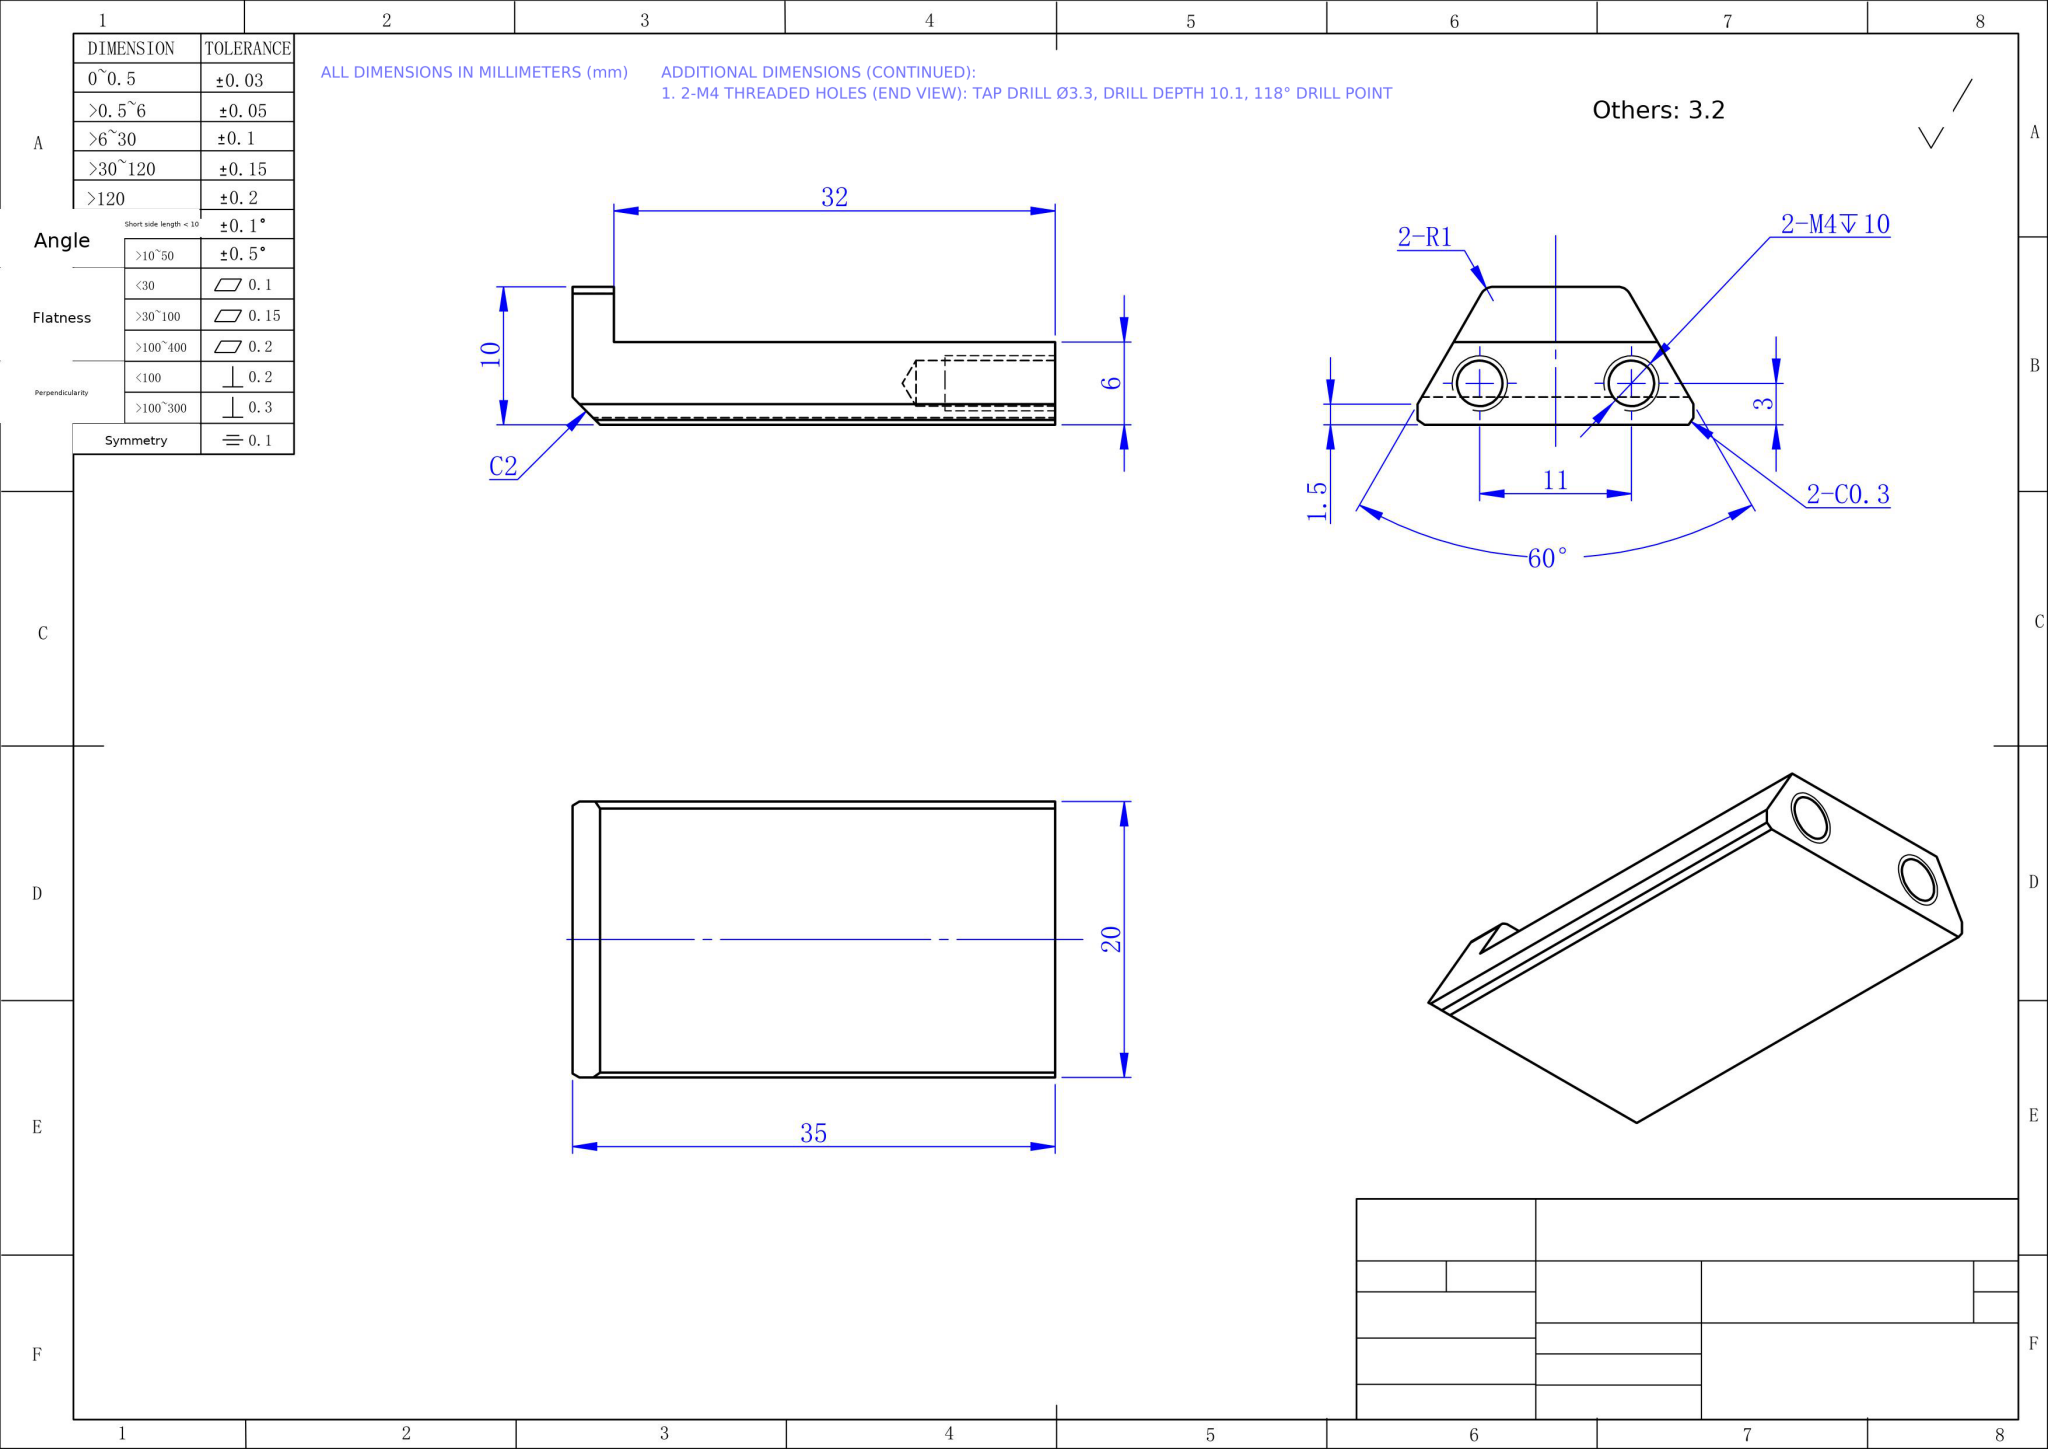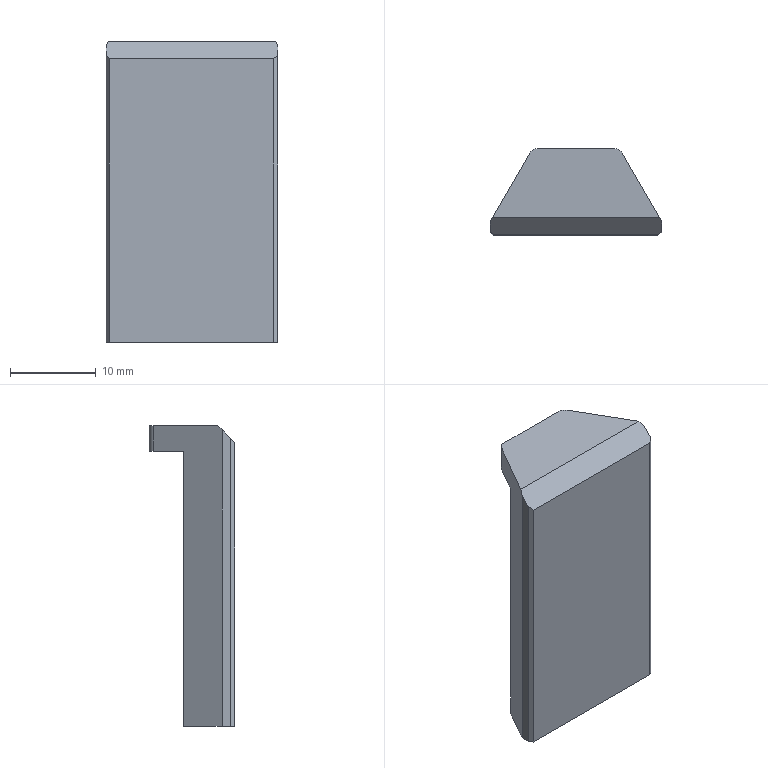Part | NX | mm | 1 solid | 23 faces | box 20 x 10 x 35 mm | volume 3716 mm3 | plane 13 | cylinder 6 | cone 4 | commonest cylinder face diameters 3.3 x4 2 x2
STEP:
#1=COLOUR_RGB('',0.7529,0.7529,0.7529);
#2=FILL_AREA_STYLE_COLOUR('',#1);
#3=FILL_AREA_STYLE('',(#2));
#4=SURFACE_STYLE_FILL_AREA(#3);
#5=SURFACE_SIDE_STYLE('',(#4));
#6=SURFACE_STYLE_USAGE(.BOTH.,#5);
#7=PRESENTATION_STYLE_ASSIGNMENT((#6));
#8=CARTESIAN_POINT('',(-3.85,3.,10.1));
#9=VERTEX_POINT('',#8);
#10=CARTESIAN_POINT('',(-7.15,3.,10.1));
#11=VERTEX_POINT('',#10);
#12=CARTESIAN_POINT('',(-5.5,3.,10.1));
#13=DIRECTION('',(0.,0.,-1.));
#14=DIRECTION('',(-1.,0.,0.));
#15=AXIS2_PLACEMENT_3D('',#12,#13,#14);
#16=CIRCLE('',#15,1.65);
#17=EDGE_CURVE('',#9,#11,#16,.T.);
#18=ORIENTED_EDGE('',*,*,#17,.F.);
#19=CARTESIAN_POINT('',(-3.85,3.,0.));
#20=VERTEX_POINT('',#19);
#21=CARTESIAN_POINT('',(-3.85,3.,0.));
#22=DIRECTION('',(0.,0.,-1.));
#23=VECTOR('',#22,1000.);
#24=LINE('',#21,#23);
#25=EDGE_CURVE('',#9,#20,#24,.T.);
#26=ORIENTED_EDGE('',*,*,#25,.T.);
#27=CARTESIAN_POINT('',(-7.15,3.,0.));
#28=VERTEX_POINT('',#27);
#29=CARTESIAN_POINT('',(-5.5,3.,0.));
#30=DIRECTION('',(0.,0.,-1.));
#31=DIRECTION('',(-1.,0.,0.));
#32=AXIS2_PLACEMENT_3D('',#29,#30,#31);
#33=CIRCLE('',#32,1.65);
#34=EDGE_CURVE('',#20,#28,#33,.T.);
#35=ORIENTED_EDGE('',*,*,#34,.T.);
#36=CARTESIAN_POINT('',(-7.15,3.,0.));
#37=DIRECTION('',(0.,0.,-1.));
#38=VECTOR('',#37,1000.);
#39=LINE('',#36,#38);
#40=EDGE_CURVE('',#11,#28,#39,.T.);
#41=ORIENTED_EDGE('',*,*,#40,.F.);
#42=EDGE_LOOP('',(#18,#26,#35,#41));
#43=FACE_OUTER_BOUND('',#42,.T.);
#44=CARTESIAN_POINT('',(-5.5,3.,0.));
#45=DIRECTION('',(0.,0.,-1.));
#46=DIRECTION('',(-1.,0.,0.));
#47=AXIS2_PLACEMENT_3D('',#44,#45,#46);
#48=CYLINDRICAL_SURFACE('',#47,1.65);
#49=ADVANCED_FACE('',(#43),#48,.F.);
#50=CARTESIAN_POINT('',(-5.5,3.,11.091));
#51=VERTEX_POINT('',#50);
#52=CARTESIAN_POINT('',(-7.15,3.,10.1));
#53=DIRECTION('',(-0.8572,0.,-0.515));
#54=VECTOR('',#53,1000.);
#55=LINE('',#52,#54);
#56=EDGE_CURVE('',#51,#11,#55,.T.);
#57=ORIENTED_EDGE('',*,*,#56,.F.);
#58=CARTESIAN_POINT('',(-3.85,3.,10.1));
#59=DIRECTION('',(0.8572,0.,-0.515));
#60=VECTOR('',#59,1000.);
#61=LINE('',#58,#60);
#62=EDGE_CURVE('',#51,#9,#61,.T.);
#63=ORIENTED_EDGE('',*,*,#62,.T.);
#64=ORIENTED_EDGE('',*,*,#17,.T.);
#65=EDGE_LOOP('',(#57,#63,#64));
#66=FACE_OUTER_BOUND('',#65,.T.);
#67=CARTESIAN_POINT('',(-5.5,3.,10.1));
#68=DIRECTION('',(0.,0.,-1.));
#69=DIRECTION('',(-1.,0.,0.));
#70=AXIS2_PLACEMENT_3D('',#67,#68,#69);
#71=CONICAL_SURFACE('',#70,1.65,1.03);
#72=ADVANCED_FACE('',(#66),#71,.F.);
#73=CARTESIAN_POINT('',(7.15,3.,10.1));
#74=VERTEX_POINT('',#73);
#75=CARTESIAN_POINT('',(3.85,3.,10.1));
#76=VERTEX_POINT('',#75);
#77=CARTESIAN_POINT('',(5.5,3.,10.1));
#78=DIRECTION('',(0.,0.,-1.));
#79=DIRECTION('',(-1.,0.,0.));
#80=AXIS2_PLACEMENT_3D('',#77,#78,#79);
#81=CIRCLE('',#80,1.65);
#82=EDGE_CURVE('',#74,#76,#81,.T.);
#83=ORIENTED_EDGE('',*,*,#82,.F.);
#84=CARTESIAN_POINT('',(7.15,3.,0.));
#85=VERTEX_POINT('',#84);
#86=CARTESIAN_POINT('',(7.15,3.,0.));
#87=DIRECTION('',(0.,0.,-1.));
#88=VECTOR('',#87,1000.);
#89=LINE('',#86,#88);
#90=EDGE_CURVE('',#74,#85,#89,.T.);
#91=ORIENTED_EDGE('',*,*,#90,.T.);
#92=CARTESIAN_POINT('',(3.85,3.,0.));
#93=VERTEX_POINT('',#92);
#94=CARTESIAN_POINT('',(5.5,3.,0.));
#95=DIRECTION('',(0.,0.,-1.));
#96=DIRECTION('',(-1.,0.,0.));
#97=AXIS2_PLACEMENT_3D('',#94,#95,#96);
#98=CIRCLE('',#97,1.65);
#99=EDGE_CURVE('',#85,#93,#98,.T.);
#100=ORIENTED_EDGE('',*,*,#99,.T.);
#101=CARTESIAN_POINT('',(3.85,3.,0.));
#102=DIRECTION('',(0.,0.,-1.));
#103=VECTOR('',#102,1000.);
#104=LINE('',#101,#103);
#105=EDGE_CURVE('',#76,#93,#104,.T.);
#106=ORIENTED_EDGE('',*,*,#105,.F.);
#107=EDGE_LOOP('',(#83,#91,#100,#106));
#108=FACE_OUTER_BOUND('',#107,.T.);
#109=CARTESIAN_POINT('',(5.5,3.,0.));
#110=DIRECTION('',(0.,0.,-1.));
#111=DIRECTION('',(-1.,0.,0.));
#112=AXIS2_PLACEMENT_3D('',#109,#110,#111);
#113=CYLINDRICAL_SURFACE('',#112,1.65);
#114=ADVANCED_FACE('',(#108),#113,.F.);
#115=CARTESIAN_POINT('',(5.5,3.,11.091));
#116=VERTEX_POINT('',#115);
#117=CARTESIAN_POINT('',(3.85,3.,10.1));
#118=DIRECTION('',(-0.8572,0.,-0.515));
#119=VECTOR('',#118,1000.);
#120=LINE('',#117,#119);
#121=EDGE_CURVE('',#116,#76,#120,.T.);
#122=ORIENTED_EDGE('',*,*,#121,.F.);
#123=CARTESIAN_POINT('',(7.15,3.,10.1));
#124=DIRECTION('',(0.8572,0.,-0.515));
#125=VECTOR('',#124,1000.);
#126=LINE('',#123,#125);
#127=EDGE_CURVE('',#116,#74,#126,.T.);
#128=ORIENTED_EDGE('',*,*,#127,.T.);
#129=ORIENTED_EDGE('',*,*,#82,.T.);
#130=EDGE_LOOP('',(#122,#128,#129));
#131=FACE_OUTER_BOUND('',#130,.T.);
#132=CARTESIAN_POINT('',(5.5,3.,10.1));
#133=DIRECTION('',(0.,0.,-1.));
#134=DIRECTION('',(-1.,0.,0.));
#135=AXIS2_PLACEMENT_3D('',#132,#133,#134);
#136=CONICAL_SURFACE('',#135,1.65,1.03);
#137=ADVANCED_FACE('',(#131),#136,.F.);
#138=CARTESIAN_POINT('',(7.402,6.,32.));
#139=VERTEX_POINT('',#138);
#140=CARTESIAN_POINT('',(-7.402,6.,32.));
#141=VERTEX_POINT('',#140);
#142=CARTESIAN_POINT('',(-7.402,6.,32.));
#143=DIRECTION('',(-1.,0.,0.));
#144=VECTOR('',#143,1000.);
#145=LINE('',#142,#144);
#146=EDGE_CURVE('',#139,#141,#145,.T.);
#147=ORIENTED_EDGE('',*,*,#146,.F.);
#148=CARTESIAN_POINT('',(7.402,6.,0.));
#149=VERTEX_POINT('',#148);
#150=CARTESIAN_POINT('',(7.402,6.,35.));
#151=DIRECTION('',(0.,0.,-1.));
#152=VECTOR('',#151,1000.);
#153=LINE('',#150,#152);
#154=EDGE_CURVE('',#139,#149,#153,.T.);
#155=ORIENTED_EDGE('',*,*,#154,.T.);
#156=CARTESIAN_POINT('',(-7.402,6.,0.));
#157=VERTEX_POINT('',#156);
#158=CARTESIAN_POINT('',(-7.402,6.,0.));
#159=DIRECTION('',(-1.,0.,0.));
#160=VECTOR('',#159,1000.);
#161=LINE('',#158,#160);
#162=EDGE_CURVE('',#149,#157,#161,.T.);
#163=ORIENTED_EDGE('',*,*,#162,.T.);
#164=CARTESIAN_POINT('',(-7.402,6.,35.));
#165=DIRECTION('',(0.,0.,-1.));
#166=VECTOR('',#165,1000.);
#167=LINE('',#164,#166);
#168=EDGE_CURVE('',#141,#157,#167,.T.);
#169=ORIENTED_EDGE('',*,*,#168,.F.);
#170=EDGE_LOOP('',(#147,#155,#163,#169));
#171=FACE_OUTER_BOUND('',#170,.T.);
#172=CARTESIAN_POINT('',(-7.402,6.,35.));
#173=DIRECTION('',(0.,-1.,0.));
#174=DIRECTION('',(0.,0.,-1.));
#175=AXIS2_PLACEMENT_3D('',#172,#173,#174);
#176=PLANE('',#175);
#177=ADVANCED_FACE('',(#171),#176,.F.);
#178=CARTESIAN_POINT('',(9.5,-0.,0.));
#179=VERTEX_POINT('',#178);
#180=CARTESIAN_POINT('',(9.5,-0.,33.));
#181=VERTEX_POINT('',#180);
#182=CARTESIAN_POINT('',(9.5,-0.,35.));
#183=DIRECTION('',(0.,0.,1.));
#184=VECTOR('',#183,1000.);
#185=LINE('',#182,#184);
#186=EDGE_CURVE('',#179,#181,#185,.T.);
#187=ORIENTED_EDGE('',*,*,#186,.T.);
#188=CARTESIAN_POINT('',(-9.65,-0.,33.));
#189=VERTEX_POINT('',#188);
#190=CARTESIAN_POINT('',(10.,-0.,33.));
#191=DIRECTION('',(-1.,0.,0.));
#192=VECTOR('',#191,1000.);
#193=LINE('',#190,#192);
#194=EDGE_CURVE('',#181,#189,#193,.T.);
#195=ORIENTED_EDGE('',*,*,#194,.T.);
#196=CARTESIAN_POINT('',(-9.65,-0.,0.));
#197=VERTEX_POINT('',#196);
#198=CARTESIAN_POINT('',(-9.65,-0.,35.));
#199=DIRECTION('',(0.,0.,-1.));
#200=VECTOR('',#199,1000.);
#201=LINE('',#198,#200);
#202=EDGE_CURVE('',#189,#197,#201,.T.);
#203=ORIENTED_EDGE('',*,*,#202,.T.);
#204=CARTESIAN_POINT('',(10.,-0.,0.));
#205=DIRECTION('',(1.,0.,0.));
#206=VECTOR('',#205,1000.);
#207=LINE('',#204,#206);
#208=EDGE_CURVE('',#197,#179,#207,.T.);
#209=ORIENTED_EDGE('',*,*,#208,.T.);
#210=EDGE_LOOP('',(#187,#195,#203,#209));
#211=FACE_OUTER_BOUND('',#210,.T.);
#212=CARTESIAN_POINT('',(10.,-0.,35.));
#213=DIRECTION('',(0.,1.,0.));
#214=DIRECTION('',(0.,0.,1.));
#215=AXIS2_PLACEMENT_3D('',#212,#213,#214);
#216=PLANE('',#215);
#217=ADVANCED_FACE('',(#211),#216,.F.);
#218=CARTESIAN_POINT('',(10.,1.5,34.5));
#219=VERTEX_POINT('',#218);
#220=CARTESIAN_POINT('',(10.,1.5,0.));
#221=VERTEX_POINT('',#220);
#222=CARTESIAN_POINT('',(10.,1.5,35.));
#223=DIRECTION('',(0.,0.,-1.));
#224=VECTOR('',#223,1000.);
#225=LINE('',#222,#224);
#226=EDGE_CURVE('',#219,#221,#225,.T.);
#227=ORIENTED_EDGE('',*,*,#226,.F.);
#228=CARTESIAN_POINT('',(10.,0.3501,33.35));
#229=VERTEX_POINT('',#228);
#230=CARTESIAN_POINT('',(10.,2.,35.));
#231=DIRECTION('',(0.,-0.7071,-0.7071));
#232=VECTOR('',#231,1000.);
#233=LINE('',#230,#232);
#234=EDGE_CURVE('',#219,#229,#233,.T.);
#235=ORIENTED_EDGE('',*,*,#234,.T.);
#236=CARTESIAN_POINT('',(10.,0.3501,0.));
#237=VERTEX_POINT('',#236);
#238=CARTESIAN_POINT('',(10.,0.3501,35.));
#239=DIRECTION('',(0.,0.,-1.));
#240=VECTOR('',#239,1000.);
#241=LINE('',#238,#240);
#242=EDGE_CURVE('',#229,#237,#241,.T.);
#243=ORIENTED_EDGE('',*,*,#242,.T.);
#244=CARTESIAN_POINT('',(10.,1.5,0.));
#245=DIRECTION('',(0.,1.,0.));
#246=VECTOR('',#245,1000.);
#247=LINE('',#244,#246);
#248=EDGE_CURVE('',#237,#221,#247,.T.);
#249=ORIENTED_EDGE('',*,*,#248,.T.);
#250=EDGE_LOOP('',(#227,#235,#243,#249));
#251=FACE_OUTER_BOUND('',#250,.T.);
#252=CARTESIAN_POINT('',(10.,1.5,35.));
#253=DIRECTION('',(-1.,0.,0.));
#254=DIRECTION('',(0.,0.,1.));
#255=AXIS2_PLACEMENT_3D('',#252,#253,#254);
#256=PLANE('',#255);
#257=ADVANCED_FACE('',(#251),#256,.F.);
#258=CARTESIAN_POINT('',(9.711,2.,35.));
#259=VERTEX_POINT('',#258);
#260=CARTESIAN_POINT('',(5.381,9.5,35.));
#261=VERTEX_POINT('',#260);
#262=CARTESIAN_POINT('',(7.402,6.,35.));
#263=DIRECTION('',(-0.5,0.866,0.));
#264=VECTOR('',#263,1000.);
#265=LINE('',#262,#264);
#266=EDGE_CURVE('',#259,#261,#265,.T.);
#267=ORIENTED_EDGE('',*,*,#266,.F.);
#268=CARTESIAN_POINT('',(8.324,4.403,37.403));
#269=DIRECTION('',(0.378,-0.6547,-0.6547));
#270=VECTOR('',#269,1000.);
#271=LINE('',#268,#270);
#272=EDGE_CURVE('',#259,#219,#271,.T.);
#273=ORIENTED_EDGE('',*,*,#272,.T.);
#274=ORIENTED_EDGE('',*,*,#226,.T.);
#275=CARTESIAN_POINT('',(7.402,6.,0.));
#276=DIRECTION('',(-0.5,0.866,0.));
#277=VECTOR('',#276,1000.);
#278=LINE('',#275,#277);
#279=EDGE_CURVE('',#221,#149,#278,.T.);
#280=ORIENTED_EDGE('',*,*,#279,.T.);
#281=ORIENTED_EDGE('',*,*,#154,.F.);
#282=CARTESIAN_POINT('',(5.381,9.5,32.));
#283=VERTEX_POINT('',#282);
#284=CARTESIAN_POINT('',(1.969,15.41,32.));
#285=DIRECTION('',(0.5,-0.866,0.));
#286=VECTOR('',#285,1000.);
#287=LINE('',#284,#286);
#288=EDGE_CURVE('',#283,#139,#287,.T.);
#289=ORIENTED_EDGE('',*,*,#288,.F.);
#290=CARTESIAN_POINT('',(5.381,9.5,35.));
#291=DIRECTION('',(0.,0.,1.));
#292=VECTOR('',#291,1000.);
#293=LINE('',#290,#292);
#294=EDGE_CURVE('',#283,#261,#293,.T.);
#295=ORIENTED_EDGE('',*,*,#294,.T.);
#296=EDGE_LOOP('',(#267,#273,#274,#280,#281,#289,#295));
#297=FACE_OUTER_BOUND('',#296,.T.);
#298=CARTESIAN_POINT('',(7.402,6.,35.));
#299=DIRECTION('',(-0.866,-0.5,0.));
#300=DIRECTION('',(0.5,-0.866,0.));
#301=AXIS2_PLACEMENT_3D('',#298,#299,#300);
#302=PLANE('',#301);
#303=ADVANCED_FACE('',(#297),#302,.F.);
#304=CARTESIAN_POINT('',(-10.,1.5,34.5));
#305=VERTEX_POINT('',#304);
#306=CARTESIAN_POINT('',(-10.,1.5,0.));
#307=VERTEX_POINT('',#306);
#308=CARTESIAN_POINT('',(-10.,1.5,35.));
#309=DIRECTION('',(0.,0.,-1.));
#310=VECTOR('',#309,1000.);
#311=LINE('',#308,#310);
#312=EDGE_CURVE('',#305,#307,#311,.T.);
#313=ORIENTED_EDGE('',*,*,#312,.F.);
#314=CARTESIAN_POINT('',(-9.711,2.,35.));
#315=VERTEX_POINT('',#314);
#316=CARTESIAN_POINT('',(-8.324,4.403,37.403));
#317=DIRECTION('',(0.378,0.6547,0.6547));
#318=VECTOR('',#317,1000.);
#319=LINE('',#316,#318);
#320=EDGE_CURVE('',#305,#315,#319,.T.);
#321=ORIENTED_EDGE('',*,*,#320,.T.);
#322=CARTESIAN_POINT('',(-5.381,9.5,35.));
#323=VERTEX_POINT('',#322);
#324=CARTESIAN_POINT('',(-10.,1.5,35.));
#325=DIRECTION('',(-0.5,-0.866,0.));
#326=VECTOR('',#325,1000.);
#327=LINE('',#324,#326);
#328=EDGE_CURVE('',#323,#315,#327,.T.);
#329=ORIENTED_EDGE('',*,*,#328,.F.);
#330=CARTESIAN_POINT('',(-5.381,9.5,32.));
#331=VERTEX_POINT('',#330);
#332=CARTESIAN_POINT('',(-5.381,9.5,32.));
#333=DIRECTION('',(0.,0.,-1.));
#334=VECTOR('',#333,1000.);
#335=LINE('',#332,#334);
#336=EDGE_CURVE('',#323,#331,#335,.T.);
#337=ORIENTED_EDGE('',*,*,#336,.T.);
#338=CARTESIAN_POINT('',(-5.67,9.,32.));
#339=DIRECTION('',(0.5,0.866,0.));
#340=VECTOR('',#339,1000.);
#341=LINE('',#338,#340);
#342=EDGE_CURVE('',#141,#331,#341,.T.);
#343=ORIENTED_EDGE('',*,*,#342,.F.);
#344=ORIENTED_EDGE('',*,*,#168,.T.);
#345=CARTESIAN_POINT('',(-10.,1.5,0.));
#346=DIRECTION('',(-0.5,-0.866,0.));
#347=VECTOR('',#346,1000.);
#348=LINE('',#345,#347);
#349=EDGE_CURVE('',#157,#307,#348,.T.);
#350=ORIENTED_EDGE('',*,*,#349,.T.);
#351=EDGE_LOOP('',(#313,#321,#329,#337,#343,#344,#350));
#352=FACE_OUTER_BOUND('',#351,.T.);
#353=CARTESIAN_POINT('',(-10.,1.5,35.));
#354=DIRECTION('',(0.866,-0.5,0.));
#355=DIRECTION('',(0.5,0.866,0.));
#356=AXIS2_PLACEMENT_3D('',#353,#354,#355);
#357=PLANE('',#356);
#358=ADVANCED_FACE('',(#352),#357,.F.);
#359=CARTESIAN_POINT('',(-10.,0.5,0.));
#360=VERTEX_POINT('',#359);
#361=CARTESIAN_POINT('',(-10.,0.5,33.5));
#362=VERTEX_POINT('',#361);
#363=CARTESIAN_POINT('',(-10.,0.5,35.));
#364=DIRECTION('',(0.,0.,1.));
#365=VECTOR('',#364,1000.);
#366=LINE('',#363,#365);
#367=EDGE_CURVE('',#360,#362,#366,.T.);
#368=ORIENTED_EDGE('',*,*,#367,.T.);
#369=CARTESIAN_POINT('',(-10.,2.,35.));
#370=DIRECTION('',(0.,0.7071,0.7071));
#371=VECTOR('',#370,1000.);
#372=LINE('',#369,#371);
#373=EDGE_CURVE('',#362,#305,#372,.T.);
#374=ORIENTED_EDGE('',*,*,#373,.T.);
#375=ORIENTED_EDGE('',*,*,#312,.T.);
#376=CARTESIAN_POINT('',(-10.,-0.,0.));
#377=DIRECTION('',(0.,-1.,0.));
#378=VECTOR('',#377,1000.);
#379=LINE('',#376,#378);
#380=EDGE_CURVE('',#307,#360,#379,.T.);
#381=ORIENTED_EDGE('',*,*,#380,.T.);
#382=EDGE_LOOP('',(#368,#374,#375,#381));
#383=FACE_OUTER_BOUND('',#382,.T.);
#384=CARTESIAN_POINT('',(-10.,-0.,35.));
#385=DIRECTION('',(1.,0.,0.));
#386=DIRECTION('',(0.,0.,-1.));
#387=AXIS2_PLACEMENT_3D('',#384,#385,#386);
#388=PLANE('',#387);
#389=ADVANCED_FACE('',(#383),#388,.F.);
#390=ORIENTED_EDGE('',*,*,#328,.T.);
#391=CARTESIAN_POINT('',(0.,2.,35.));
#392=DIRECTION('',(1.,0.,0.));
#393=VECTOR('',#392,1000.);
#394=LINE('',#391,#393);
#395=EDGE_CURVE('',#315,#259,#394,.T.);
#396=ORIENTED_EDGE('',*,*,#395,.T.);
#397=ORIENTED_EDGE('',*,*,#266,.T.);
#398=CARTESIAN_POINT('',(4.515,10.,35.));
#399=VERTEX_POINT('',#398);
#400=CARTESIAN_POINT('',(4.515,9.,35.));
#401=DIRECTION('',(0.,0.,1.));
#402=DIRECTION('',(-1.,0.,0.));
#403=AXIS2_PLACEMENT_3D('',#400,#401,#402);
#404=CIRCLE('',#403,1.);
#405=EDGE_CURVE('',#261,#399,#404,.T.);
#406=ORIENTED_EDGE('',*,*,#405,.T.);
#407=CARTESIAN_POINT('',(-4.515,10.,35.));
#408=VERTEX_POINT('',#407);
#409=CARTESIAN_POINT('',(-7.402,10.,35.));
#410=DIRECTION('',(1.,0.,0.));
#411=VECTOR('',#410,1000.);
#412=LINE('',#409,#411);
#413=EDGE_CURVE('',#408,#399,#412,.T.);
#414=ORIENTED_EDGE('',*,*,#413,.F.);
#415=CARTESIAN_POINT('',(-4.515,9.,35.));
#416=DIRECTION('',(0.,0.,1.));
#417=DIRECTION('',(-1.,-0.,0.));
#418=AXIS2_PLACEMENT_3D('',#415,#416,#417);
#419=CIRCLE('',#418,1.);
#420=EDGE_CURVE('',#408,#323,#419,.T.);
#421=ORIENTED_EDGE('',*,*,#420,.T.);
#422=EDGE_LOOP('',(#390,#396,#397,#406,#414,#421));
#423=FACE_OUTER_BOUND('',#422,.T.);
#424=CARTESIAN_POINT('',(0.,0.,35.));
#425=DIRECTION('',(0.,0.,-1.));
#426=DIRECTION('',(-1.,0.,0.));
#427=AXIS2_PLACEMENT_3D('',#424,#425,#426);
#428=PLANE('',#427);
#429=ADVANCED_FACE('',(#423),#428,.F.);
#430=CARTESIAN_POINT('',(-5.5,3.,0.));
#431=DIRECTION('',(0.,0.,-1.));
#432=DIRECTION('',(-1.,0.,0.));
#433=AXIS2_PLACEMENT_3D('',#430,#431,#432);
#434=CIRCLE('',#433,1.65);
#435=EDGE_CURVE('',#28,#20,#434,.T.);
#436=ORIENTED_EDGE('',*,*,#435,.F.);
#437=ORIENTED_EDGE('',*,*,#34,.F.);
#438=EDGE_LOOP('',(#436,#437));
#439=FACE_BOUND('',#438,.T.);
#440=CARTESIAN_POINT('',(5.5,3.,0.));
#441=DIRECTION('',(0.,0.,-1.));
#442=DIRECTION('',(-1.,0.,0.));
#443=AXIS2_PLACEMENT_3D('',#440,#441,#442);
#444=CIRCLE('',#443,1.65);
#445=EDGE_CURVE('',#93,#85,#444,.T.);
#446=ORIENTED_EDGE('',*,*,#445,.F.);
#447=ORIENTED_EDGE('',*,*,#99,.F.);
#448=EDGE_LOOP('',(#446,#447));
#449=FACE_BOUND('',#448,.T.);
#450=ORIENTED_EDGE('',*,*,#208,.F.);
#451=CARTESIAN_POINT('',(-6.475,-4.534,0.));
#452=DIRECTION('',(-0.5736,0.8192,0.));
#453=VECTOR('',#452,1000.);
#454=LINE('',#451,#453);
#455=EDGE_CURVE('',#197,#360,#454,.T.);
#456=ORIENTED_EDGE('',*,*,#455,.T.);
#457=ORIENTED_EDGE('',*,*,#380,.F.);
#458=ORIENTED_EDGE('',*,*,#349,.F.);
#459=ORIENTED_EDGE('',*,*,#162,.F.);
#460=ORIENTED_EDGE('',*,*,#279,.F.);
#461=ORIENTED_EDGE('',*,*,#248,.F.);
#462=CARTESIAN_POINT('',(3.125,-4.464,0.));
#463=DIRECTION('',(-0.8192,-0.5736,0.));
#464=VECTOR('',#463,1000.);
#465=LINE('',#462,#464);
#466=EDGE_CURVE('',#237,#179,#465,.T.);
#467=ORIENTED_EDGE('',*,*,#466,.T.);
#468=EDGE_LOOP('',(#450,#456,#457,#458,#459,#460,#461,#467));
#469=FACE_OUTER_BOUND('',#468,.T.);
#470=CARTESIAN_POINT('',(0.,0.,0.));
#471=DIRECTION('',(0.,0.,-1.));
#472=DIRECTION('',(-1.,0.,0.));
#473=AXIS2_PLACEMENT_3D('',#470,#471,#472);
#474=PLANE('',#473);
#475=ADVANCED_FACE('',(#439,#449,#469),#474,.T.);
#476=ORIENTED_EDGE('',*,*,#342,.T.);
#477=CARTESIAN_POINT('',(-4.515,10.,32.));
#478=VERTEX_POINT('',#477);
#479=CARTESIAN_POINT('',(-4.515,9.,32.));
#480=DIRECTION('',(0.,0.,-1.));
#481=DIRECTION('',(1.,-0.,0.));
#482=AXIS2_PLACEMENT_3D('',#479,#480,#481);
#483=CIRCLE('',#482,1.);
#484=EDGE_CURVE('',#331,#478,#483,.T.);
#485=ORIENTED_EDGE('',*,*,#484,.T.);
#486=CARTESIAN_POINT('',(4.515,10.,32.));
#487=VERTEX_POINT('',#486);
#488=CARTESIAN_POINT('',(-7.402,10.,32.));
#489=DIRECTION('',(-1.,0.,0.));
#490=VECTOR('',#489,1000.);
#491=LINE('',#488,#490);
#492=EDGE_CURVE('',#487,#478,#491,.T.);
#493=ORIENTED_EDGE('',*,*,#492,.F.);
#494=CARTESIAN_POINT('',(4.515,9.,32.));
#495=DIRECTION('',(0.,0.,-1.));
#496=DIRECTION('',(1.,0.,0.));
#497=AXIS2_PLACEMENT_3D('',#494,#495,#496);
#498=CIRCLE('',#497,1.);
#499=EDGE_CURVE('',#487,#283,#498,.T.);
#500=ORIENTED_EDGE('',*,*,#499,.T.);
#501=ORIENTED_EDGE('',*,*,#288,.T.);
#502=ORIENTED_EDGE('',*,*,#146,.T.);
#503=EDGE_LOOP('',(#476,#485,#493,#500,#501,#502));
#504=FACE_OUTER_BOUND('',#503,.T.);
#505=CARTESIAN_POINT('',(-7.402,10.,32.));
#506=DIRECTION('',(0.,0.,1.));
#507=DIRECTION('',(1.,0.,0.));
#508=AXIS2_PLACEMENT_3D('',#505,#506,#507);
#509=PLANE('',#508);
#510=ADVANCED_FACE('',(#504),#509,.F.);
#511=ORIENTED_EDGE('',*,*,#492,.T.);
#512=CARTESIAN_POINT('',(-4.515,10.,35.));
#513=DIRECTION('',(0.,0.,1.));
#514=VECTOR('',#513,1000.);
#515=LINE('',#512,#514);
#516=EDGE_CURVE('',#478,#408,#515,.T.);
#517=ORIENTED_EDGE('',*,*,#516,.T.);
#518=ORIENTED_EDGE('',*,*,#413,.T.);
#519=CARTESIAN_POINT('',(4.515,10.,32.));
#520=DIRECTION('',(0.,0.,-1.));
#521=VECTOR('',#520,1000.);
#522=LINE('',#519,#521);
#523=EDGE_CURVE('',#399,#487,#522,.T.);
#524=ORIENTED_EDGE('',*,*,#523,.T.);
#525=EDGE_LOOP('',(#511,#517,#518,#524));
#526=FACE_OUTER_BOUND('',#525,.T.);
#527=CARTESIAN_POINT('',(0.,10.,0.));
#528=DIRECTION('',(0.,1.,0.));
#529=DIRECTION('',(0.,0.,1.));
#530=AXIS2_PLACEMENT_3D('',#527,#528,#529);
#531=PLANE('',#530);
#532=ADVANCED_FACE('',(#526),#531,.T.);
#533=ORIENTED_EDGE('',*,*,#127,.F.);
#534=ORIENTED_EDGE('',*,*,#121,.T.);
#535=CARTESIAN_POINT('',(5.5,3.,10.1));
#536=DIRECTION('',(0.,0.,-1.));
#537=DIRECTION('',(-1.,0.,0.));
#538=AXIS2_PLACEMENT_3D('',#535,#536,#537);
#539=CIRCLE('',#538,1.65);
#540=EDGE_CURVE('',#76,#74,#539,.T.);
#541=ORIENTED_EDGE('',*,*,#540,.T.);
#542=EDGE_LOOP('',(#533,#534,#541));
#543=FACE_OUTER_BOUND('',#542,.T.);
#544=CARTESIAN_POINT('',(5.5,3.,10.1));
#545=DIRECTION('',(0.,0.,-1.));
#546=DIRECTION('',(-1.,0.,0.));
#547=AXIS2_PLACEMENT_3D('',#544,#545,#546);
#548=CONICAL_SURFACE('',#547,1.65,1.03);
#549=ADVANCED_FACE('',(#543),#548,.F.);
#550=ORIENTED_EDGE('',*,*,#90,.F.);
#551=ORIENTED_EDGE('',*,*,#540,.F.);
#552=ORIENTED_EDGE('',*,*,#105,.T.);
#553=ORIENTED_EDGE('',*,*,#445,.T.);
#554=EDGE_LOOP('',(#550,#551,#552,#553));
#555=FACE_OUTER_BOUND('',#554,.T.);
#556=CARTESIAN_POINT('',(5.5,3.,0.));
#557=DIRECTION('',(0.,0.,-1.));
#558=DIRECTION('',(-1.,0.,0.));
#559=AXIS2_PLACEMENT_3D('',#556,#557,#558);
#560=CYLINDRICAL_SURFACE('',#559,1.65);
#561=ADVANCED_FACE('',(#555),#560,.F.);
#562=ORIENTED_EDGE('',*,*,#62,.F.);
#563=ORIENTED_EDGE('',*,*,#56,.T.);
#564=CARTESIAN_POINT('',(-5.5,3.,10.1));
#565=DIRECTION('',(0.,0.,-1.));
#566=DIRECTION('',(-1.,0.,0.));
#567=AXIS2_PLACEMENT_3D('',#564,#565,#566);
#568=CIRCLE('',#567,1.65);
#569=EDGE_CURVE('',#11,#9,#568,.T.);
#570=ORIENTED_EDGE('',*,*,#569,.T.);
#571=EDGE_LOOP('',(#562,#563,#570));
#572=FACE_OUTER_BOUND('',#571,.T.);
#573=CARTESIAN_POINT('',(-5.5,3.,10.1));
#574=DIRECTION('',(0.,0.,-1.));
#575=DIRECTION('',(-1.,0.,0.));
#576=AXIS2_PLACEMENT_3D('',#573,#574,#575);
#577=CONICAL_SURFACE('',#576,1.65,1.03);
#578=ADVANCED_FACE('',(#572),#577,.F.);
#579=ORIENTED_EDGE('',*,*,#25,.F.);
#580=ORIENTED_EDGE('',*,*,#569,.F.);
#581=ORIENTED_EDGE('',*,*,#40,.T.);
#582=ORIENTED_EDGE('',*,*,#435,.T.);
#583=EDGE_LOOP('',(#579,#580,#581,#582));
#584=FACE_OUTER_BOUND('',#583,.T.);
#585=CARTESIAN_POINT('',(-5.5,3.,0.));
#586=DIRECTION('',(0.,0.,-1.));
#587=DIRECTION('',(-1.,0.,0.));
#588=AXIS2_PLACEMENT_3D('',#585,#586,#587);
#589=CYLINDRICAL_SURFACE('',#588,1.65);
#590=ADVANCED_FACE('',(#584),#589,.F.);
#591=ORIENTED_EDGE('',*,*,#202,.F.);
#592=CARTESIAN_POINT('',(-10.212,0.8031,33.803));
#593=DIRECTION('',(-0.4437,0.6337,0.6337));
#594=VECTOR('',#593,1000.);
#595=LINE('',#592,#594);
#596=EDGE_CURVE('',#189,#362,#595,.T.);
#597=ORIENTED_EDGE('',*,*,#596,.T.);
#598=ORIENTED_EDGE('',*,*,#367,.F.);
#599=ORIENTED_EDGE('',*,*,#455,.F.);
#600=EDGE_LOOP('',(#591,#597,#598,#599));
#601=FACE_OUTER_BOUND('',#600,.T.);
#602=CARTESIAN_POINT('',(-9.65,-0.,35.));
#603=DIRECTION('',(0.8192,0.5736,0.));
#604=DIRECTION('',(0.,0.,-1.));
#605=AXIS2_PLACEMENT_3D('',#602,#603,#604);
#606=PLANE('',#605);
#607=ADVANCED_FACE('',(#601),#606,.F.);
#608=ORIENTED_EDGE('',*,*,#242,.F.);
#609=CARTESIAN_POINT('',(10.583,0.7585,33.759));
#610=DIRECTION('',(-0.7106,-0.4975,-0.4975));
#611=VECTOR('',#610,1000.);
#612=LINE('',#609,#611);
#613=EDGE_CURVE('',#229,#181,#612,.T.);
#614=ORIENTED_EDGE('',*,*,#613,.T.);
#615=ORIENTED_EDGE('',*,*,#186,.F.);
#616=ORIENTED_EDGE('',*,*,#466,.F.);
#617=EDGE_LOOP('',(#608,#614,#615,#616));
#618=FACE_OUTER_BOUND('',#617,.T.);
#619=CARTESIAN_POINT('',(10.,0.3501,35.));
#620=DIRECTION('',(-0.5736,0.8192,0.));
#621=DIRECTION('',(0.,0.,-1.));
#622=AXIS2_PLACEMENT_3D('',#619,#620,#621);
#623=PLANE('',#622);
#624=ADVANCED_FACE('',(#618),#623,.F.);
#625=ORIENTED_EDGE('',*,*,#484,.F.);
#626=ORIENTED_EDGE('',*,*,#336,.F.);
#627=ORIENTED_EDGE('',*,*,#420,.F.);
#628=ORIENTED_EDGE('',*,*,#516,.F.);
#629=EDGE_LOOP('',(#625,#626,#627,#628));
#630=FACE_OUTER_BOUND('',#629,.T.);
#631=CARTESIAN_POINT('',(-4.515,9.,0.));
#632=DIRECTION('',(0.,0.,-1.));
#633=DIRECTION('',(-1.,0.,0.));
#634=AXIS2_PLACEMENT_3D('',#631,#632,#633);
#635=CYLINDRICAL_SURFACE('',#634,1.);
#636=ADVANCED_FACE('',(#630),#635,.T.);
#637=ORIENTED_EDGE('',*,*,#499,.F.);
#638=ORIENTED_EDGE('',*,*,#523,.F.);
#639=ORIENTED_EDGE('',*,*,#405,.F.);
#640=ORIENTED_EDGE('',*,*,#294,.F.);
#641=EDGE_LOOP('',(#637,#638,#639,#640));
#642=FACE_OUTER_BOUND('',#641,.T.);
#643=CARTESIAN_POINT('',(4.515,9.,35.));
#644=DIRECTION('',(0.,0.,-1.));
#645=DIRECTION('',(-1.,0.,0.));
#646=AXIS2_PLACEMENT_3D('',#643,#644,#645);
#647=CYLINDRICAL_SURFACE('',#646,1.);
#648=ADVANCED_FACE('',(#642),#647,.T.);
#649=ORIENTED_EDGE('',*,*,#596,.F.);
#650=ORIENTED_EDGE('',*,*,#194,.F.);
#651=ORIENTED_EDGE('',*,*,#613,.F.);
#652=ORIENTED_EDGE('',*,*,#234,.F.);
#653=ORIENTED_EDGE('',*,*,#272,.F.);
#654=ORIENTED_EDGE('',*,*,#395,.F.);
#655=ORIENTED_EDGE('',*,*,#320,.F.);
#656=ORIENTED_EDGE('',*,*,#373,.F.);
#657=EDGE_LOOP('',(#649,#650,#651,#652,#653,#654,#655,#656));
#658=FACE_OUTER_BOUND('',#657,.T.);
#659=CARTESIAN_POINT('',(0.,2.,35.));
#660=DIRECTION('',(0.,0.7071,-0.7071));
#661=DIRECTION('',(1.,0.,0.));
#662=AXIS2_PLACEMENT_3D('',#659,#660,#661);
#663=PLANE('',#662);
#664=ADVANCED_FACE('',(#658),#663,.F.);
#665=CLOSED_SHELL('',(#49,#72,#114,#137,#177,#217,#257,#303,#358,#389,#429,#475,#510,#532,#549,#561,#578,#590,#607,#624,#636,#648,#664));
#666=MANIFOLD_SOLID_BREP('',#665);
#667=CARTESIAN_POINT('',(0.,0.,0.));
#668=DIRECTION('',(0.,0.,1.));
#669=DIRECTION('',(1.,0.,0.));
#670=AXIS2_PLACEMENT_3D('',#667,#668,#669);
#671=(LENGTH_UNIT()NAMED_UNIT(*)SI_UNIT(.MILLI.,.METRE.));
#672=UNCERTAINTY_MEASURE_WITH_UNIT(LENGTH_MEASURE(0.00001),#671,'','');
#673=(NAMED_UNIT(*)PLANE_ANGLE_UNIT()SI_UNIT($,.RADIAN.));
#674=(NAMED_UNIT(*)SI_UNIT($,.STERADIAN.)SOLID_ANGLE_UNIT());
#675=(GEOMETRIC_REPRESENTATION_CONTEXT(3)GLOBAL_UNCERTAINTY_ASSIGNED_CONTEXT((#672))GLOBAL_UNIT_ASSIGNED_CONTEXT((#671,#673,#674))REPRESENTATION_CONTEXT('',''));
#676=ADVANCED_BREP_SHAPE_REPRESENTATION('',(#666,#670),#675);
#677=STYLED_ITEM('',(#7),#676);
#678=(LENGTH_UNIT()NAMED_UNIT(*)SI_UNIT(.MILLI.,.METRE.));
#679=UNCERTAINTY_MEASURE_WITH_UNIT(LENGTH_MEASURE(0.00001),#678,'','');
#680=(NAMED_UNIT(*)PLANE_ANGLE_UNIT()SI_UNIT($,.RADIAN.));
#681=(NAMED_UNIT(*)SI_UNIT($,.STERADIAN.)SOLID_ANGLE_UNIT());
#682=(GEOMETRIC_REPRESENTATION_CONTEXT(3)GLOBAL_UNCERTAINTY_ASSIGNED_CONTEXT((#679))GLOBAL_UNIT_ASSIGNED_CONTEXT((#678,#680,#681))REPRESENTATION_CONTEXT('',''));
#683=MECHANICAL_DESIGN_GEOMETRIC_PRESENTATION_REPRESENTATION('',(#677),#682);
#684=COLOUR_RGB('',0.7529,0.7529,0.7529);
#685=FILL_AREA_STYLE_COLOUR('',#684);
#686=FILL_AREA_STYLE('',(#685));
#687=SURFACE_STYLE_FILL_AREA(#686);
#688=SURFACE_SIDE_STYLE('',(#687));
#689=SURFACE_STYLE_USAGE(.BOTH.,#688);
#690=PRESENTATION_STYLE_ASSIGNMENT((#689));
#691=STYLED_ITEM('',(#690),#666);
#692=PRESENTATION_LAYER_ASSIGNMENT('','',(#691));
#693=PRESENTATION_LAYER_ASSIGNMENT('','',(#677));
#694=COLOUR_RGB('',0.7529,0.7529,0.7529);
#695=FILL_AREA_STYLE_COLOUR('',#694);
#696=FILL_AREA_STYLE('',(#695));
#697=SURFACE_STYLE_FILL_AREA(#696);
#698=SURFACE_SIDE_STYLE('',(#697));
#699=SURFACE_STYLE_USAGE(.BOTH.,#698);
#700=PRESENTATION_STYLE_ASSIGNMENT((#699));
#701=STYLED_ITEM('',(#700),#114);
#702=(LENGTH_UNIT()NAMED_UNIT(*)SI_UNIT(.MILLI.,.METRE.));
#703=UNCERTAINTY_MEASURE_WITH_UNIT(LENGTH_MEASURE(0.00001),#702,'','');
#704=(NAMED_UNIT(*)PLANE_ANGLE_UNIT()SI_UNIT($,.RADIAN.));
#705=(NAMED_UNIT(*)SI_UNIT($,.STERADIAN.)SOLID_ANGLE_UNIT());
#706=(GEOMETRIC_REPRESENTATION_CONTEXT(3)GLOBAL_UNCERTAINTY_ASSIGNED_CONTEXT((#703))GLOBAL_UNIT_ASSIGNED_CONTEXT((#702,#704,#705))REPRESENTATION_CONTEXT('',''));
#707=MECHANICAL_DESIGN_GEOMETRIC_PRESENTATION_REPRESENTATION('',(#701),#706);
#708=COLOUR_RGB('',0.7529,0.7529,0.7529);
#709=FILL_AREA_STYLE_COLOUR('',#708);
#710=FILL_AREA_STYLE('',(#709));
#711=SURFACE_STYLE_FILL_AREA(#710);
#712=SURFACE_SIDE_STYLE('',(#711));
#713=SURFACE_STYLE_USAGE(.BOTH.,#712);
#714=PRESENTATION_STYLE_ASSIGNMENT((#713));
#715=STYLED_ITEM('',(#714),#561);
#716=PRESENTATION_LAYER_ASSIGNMENT('','',(#715));
#717=COLOUR_RGB('',0.7529,0.7529,0.7529);
#718=FILL_AREA_STYLE_COLOUR('',#717);
#719=FILL_AREA_STYLE('',(#718));
#720=SURFACE_STYLE_FILL_AREA(#719);
#721=SURFACE_SIDE_STYLE('',(#720));
#722=SURFACE_STYLE_USAGE(.BOTH.,#721);
#723=PRESENTATION_STYLE_ASSIGNMENT((#722));
#724=STYLED_ITEM('',(#723),#49);
#725=(LENGTH_UNIT()NAMED_UNIT(*)SI_UNIT(.MILLI.,.METRE.));
#726=UNCERTAINTY_MEASURE_WITH_UNIT(LENGTH_MEASURE(0.00001),#725,'','');
#727=(NAMED_UNIT(*)PLANE_ANGLE_UNIT()SI_UNIT($,.RADIAN.));
#728=(NAMED_UNIT(*)SI_UNIT($,.STERADIAN.)SOLID_ANGLE_UNIT());
#729=(GEOMETRIC_REPRESENTATION_CONTEXT(3)GLOBAL_UNCERTAINTY_ASSIGNED_CONTEXT((#726))GLOBAL_UNIT_ASSIGNED_CONTEXT((#725,#727,#728))REPRESENTATION_CONTEXT('',''));
#730=MECHANICAL_DESIGN_GEOMETRIC_PRESENTATION_REPRESENTATION('',(#724),#729);
#731=PRESENTATION_LAYER_ASSIGNMENT('','',(#724));
#732=(LENGTH_UNIT()NAMED_UNIT(*)SI_UNIT(.MILLI.,.METRE.));
#733=UNCERTAINTY_MEASURE_WITH_UNIT(LENGTH_MEASURE(0.00001),#732,'','');
#734=(NAMED_UNIT(*)PLANE_ANGLE_UNIT()SI_UNIT($,.RADIAN.));
#735=(NAMED_UNIT(*)SI_UNIT($,.STERADIAN.)SOLID_ANGLE_UNIT());
#736=(GEOMETRIC_REPRESENTATION_CONTEXT(3)GLOBAL_UNCERTAINTY_ASSIGNED_CONTEXT((#733))GLOBAL_UNIT_ASSIGNED_CONTEXT((#732,#734,#735))REPRESENTATION_CONTEXT('',''));
#737=MECHANICAL_DESIGN_GEOMETRIC_PRESENTATION_REPRESENTATION('',(#715),#736);
#738=COLOUR_RGB('',0.7529,0.7529,0.7529);
#739=FILL_AREA_STYLE_COLOUR('',#738);
#740=FILL_AREA_STYLE('',(#739));
#741=SURFACE_STYLE_FILL_AREA(#740);
#742=SURFACE_SIDE_STYLE('',(#741));
#743=SURFACE_STYLE_USAGE(.BOTH.,#742);
#744=PRESENTATION_STYLE_ASSIGNMENT((#743));
#745=STYLED_ITEM('',(#744),#590);
#746=(LENGTH_UNIT()NAMED_UNIT(*)SI_UNIT(.MILLI.,.METRE.));
#747=UNCERTAINTY_MEASURE_WITH_UNIT(LENGTH_MEASURE(0.00001),#746,'','');
#748=(NAMED_UNIT(*)PLANE_ANGLE_UNIT()SI_UNIT($,.RADIAN.));
#749=(NAMED_UNIT(*)SI_UNIT($,.STERADIAN.)SOLID_ANGLE_UNIT());
#750=(GEOMETRIC_REPRESENTATION_CONTEXT(3)GLOBAL_UNCERTAINTY_ASSIGNED_CONTEXT((#747))GLOBAL_UNIT_ASSIGNED_CONTEXT((#746,#748,#749))REPRESENTATION_CONTEXT('',''));
#751=MECHANICAL_DESIGN_GEOMETRIC_PRESENTATION_REPRESENTATION('',(#745),#750);
#752=PRESENTATION_LAYER_ASSIGNMENT('','',(#701));
#753=(LENGTH_UNIT()NAMED_UNIT(*)SI_UNIT(.MILLI.,.METRE.));
#754=UNCERTAINTY_MEASURE_WITH_UNIT(LENGTH_MEASURE(0.00001),#753,'','');
#755=(NAMED_UNIT(*)PLANE_ANGLE_UNIT()SI_UNIT($,.RADIAN.));
#756=(NAMED_UNIT(*)SI_UNIT($,.STERADIAN.)SOLID_ANGLE_UNIT());
#757=(GEOMETRIC_REPRESENTATION_CONTEXT(3)GLOBAL_UNCERTAINTY_ASSIGNED_CONTEXT((#754))GLOBAL_UNIT_ASSIGNED_CONTEXT((#753,#755,#756))REPRESENTATION_CONTEXT('',''));
#758=MECHANICAL_DESIGN_GEOMETRIC_PRESENTATION_REPRESENTATION('',(#691),#757);
#759=PRESENTATION_LAYER_ASSIGNMENT('','',(#745));